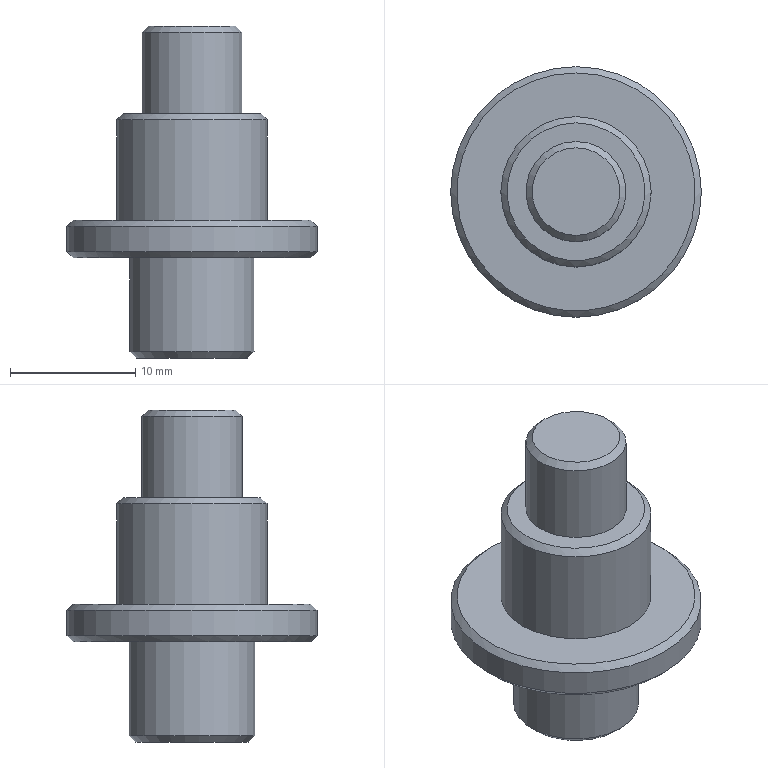Component | NX | SUPPORT_SHAFT | 1 solid | 14 faces | box 20 x 20 x 26.5 mm | volume 2857 mm3 | plane 5 | cone 5 | cylinder 4 | commonest cylinder face diameters 8 x1 12 x1 20 x1 10 x1
STEP:
#1=CARTESIAN_POINT('',(0.,0.,0.));
#2=DIRECTION('',(0.,0.,1.));
#3=DIRECTION('',(1.,0.,0.));
#4=AXIS2_PLACEMENT_3D('',#1,#2,#3);
#5=CARTESIAN_POINT('',(0.,3.5,3.5));
#6=VERTEX_POINT('',#5);
#7=CARTESIAN_POINT('',(0.,0.,3.5));
#8=DIRECTION('',(0.,0.,1.));
#9=DIRECTION('',(0.,1.,0.));
#10=AXIS2_PLACEMENT_3D('',#7,#8,#9);
#11=CIRCLE('',#10,3.5);
#12=CARTESIAN_POINT('',(0.,-4.,3.5));
#13=DIRECTION('',(0.,0.,-1.));
#14=DIRECTION('',(0.,1.,0.));
#15=AXIS2_PLACEMENT_3D('',#12,#13,#14);
#16=PLANE('',#15);
#17=CARTESIAN_POINT('',(7.5,0.));
#18=CARTESIAN_POINT('',(7.5,-6.062));
#19=CARTESIAN_POINT('',(2.25,-3.031));
#20=CARTESIAN_POINT('',(-3.,-0.));
#21=CARTESIAN_POINT('',(2.25,3.031));
#22=CARTESIAN_POINT('',(7.5,6.062));
#23=CARTESIAN_POINT('',(7.5,0.));
#24=(BOUNDED_CURVE()B_SPLINE_CURVE(2,(#17,#18,#19,#20,#21,#22,#23),.UNSPECIFIED.,.T.,.F.)B_SPLINE_CURVE_WITH_KNOTS((1,2,2,2,2,1),(-2.094,0.,2.094,4.189,6.283,8.378),.UNSPECIFIED.)CURVE()GEOMETRIC_REPRESENTATION_ITEM()RATIONAL_B_SPLINE_CURVE((1.,0.5,1.,0.5,1.,0.5,1.))REPRESENTATION_ITEM(''));
#25=(GEOMETRIC_REPRESENTATION_CONTEXT(2)PARAMETRIC_REPRESENTATION_CONTEXT()REPRESENTATION_CONTEXT('',''));
#26=DEFINITIONAL_REPRESENTATION('',(#24),#25);
#27=PCURVE('',#16,#26);
#28=CARTESIAN_POINT('',(0.,0.,3.5));
#29=DIRECTION('',(0.,0.,-1.));
#30=DIRECTION('',(0.,1.,0.));
#31=AXIS2_PLACEMENT_3D('',#28,#29,#30);
#32=CONICAL_SURFACE('',#31,3.5,0.7854);
#33=CARTESIAN_POINT('',(6.283,0.));
#34=DIRECTION('',(-1.,0.));
#35=VECTOR('',#34,1.);
#36=LINE('',#33,#35);
#37=(GEOMETRIC_REPRESENTATION_CONTEXT(2)PARAMETRIC_REPRESENTATION_CONTEXT()REPRESENTATION_CONTEXT('',''));
#38=DEFINITIONAL_REPRESENTATION('',(#36),#37);
#39=PCURVE('',#32,#38);
#40=SURFACE_CURVE('',#11,(#27,#39),.PCURVE_S1.);
#41=EDGE_CURVE('',#6,#6,#40,.T.);
#42=ORIENTED_EDGE('',*,*,#41,.T.);
#43=EDGE_LOOP('',(#42));
#44=FACE_BOUND('',#43,.T.);
#45=ADVANCED_FACE('',(#44),#16,.F.);
#46=CARTESIAN_POINT('',(0.,4.,3.));
#47=VERTEX_POINT('',#46);
#48=CARTESIAN_POINT('',(0.,-4.,3.));
#49=VERTEX_POINT('',#48);
#50=CARTESIAN_POINT('',(0.,0.,3.));
#51=DIRECTION('',(0.,0.,-1.));
#52=DIRECTION('',(0.,1.,0.));
#53=AXIS2_PLACEMENT_3D('',#50,#51,#52);
#54=CIRCLE('',#53,4.);
#55=CARTESIAN_POINT('',(0.,0.,-23.));
#56=DIRECTION('',(0.,0.,1.));
#57=DIRECTION('',(0.,-1.,0.));
#58=AXIS2_PLACEMENT_3D('',#55,#56,#57);
#59=CYLINDRICAL_SURFACE('',#58,4.);
#60=CARTESIAN_POINT('',(3.142,26.));
#61=DIRECTION('',(-1.,0.));
#62=VECTOR('',#61,1.);
#63=LINE('',#60,#62);
#64=(GEOMETRIC_REPRESENTATION_CONTEXT(2)PARAMETRIC_REPRESENTATION_CONTEXT()REPRESENTATION_CONTEXT('',''));
#65=DEFINITIONAL_REPRESENTATION('',(#63),#64);
#66=PCURVE('',#59,#65);
#67=CARTESIAN_POINT('',(0.,0.5));
#68=DIRECTION('',(1.,0.));
#69=VECTOR('',#68,1.);
#70=LINE('',#67,#69);
#71=(GEOMETRIC_REPRESENTATION_CONTEXT(2)PARAMETRIC_REPRESENTATION_CONTEXT()REPRESENTATION_CONTEXT('',''));
#72=DEFINITIONAL_REPRESENTATION('',(#70),#71);
#73=PCURVE('',#32,#72);
#74=SURFACE_CURVE('',#54,(#66,#73),.PCURVE_S1.);
#75=EDGE_CURVE('',#47,#49,#74,.T.);
#76=ORIENTED_EDGE('',*,*,#75,.T.);
#77=CARTESIAN_POINT('',(0.,-4.,-3.5));
#78=VERTEX_POINT('',#77);
#79=CARTESIAN_POINT('',(0.,-4.,-3.5));
#80=CARTESIAN_POINT('',(0.,-4.,3.));
#81=B_SPLINE_CURVE_WITH_KNOTS('',1,(#79,#80),.UNSPECIFIED.,.F.,.F.,(2,2),(19.5,26.),.PIECEWISE_BEZIER_KNOTS.);
#82=CARTESIAN_POINT('',(0.,0.));
#83=DIRECTION('',(0.,1.));
#84=VECTOR('',#83,1.);
#85=LINE('',#82,#84);
#86=(GEOMETRIC_REPRESENTATION_CONTEXT(2)PARAMETRIC_REPRESENTATION_CONTEXT()REPRESENTATION_CONTEXT('',''));
#87=DEFINITIONAL_REPRESENTATION('',(#85),#86);
#88=PCURVE('',#59,#87);
#89=CARTESIAN_POINT('',(6.283,0.));
#90=DIRECTION('',(0.,1.));
#91=VECTOR('',#90,1.);
#92=LINE('',#89,#91);
#93=(GEOMETRIC_REPRESENTATION_CONTEXT(2)PARAMETRIC_REPRESENTATION_CONTEXT()REPRESENTATION_CONTEXT('',''));
#94=DEFINITIONAL_REPRESENTATION('',(#92),#93);
#95=PCURVE('',#59,#94);
#96=SEAM_CURVE('',#81,(#88,#95),.PCURVE_S1.);
#97=EDGE_CURVE('',#78,#49,#96,.T.);
#98=ORIENTED_EDGE('',*,*,#97,.F.);
#99=CARTESIAN_POINT('',(0.,0.,-3.5));
#100=DIRECTION('',(0.,0.,1.));
#101=DIRECTION('',(0.,-1.,0.));
#102=AXIS2_PLACEMENT_3D('',#99,#100,#101);
#103=CIRCLE('',#102,4.);
#104=CARTESIAN_POINT('',(0.,19.5));
#105=DIRECTION('',(1.,0.));
#106=VECTOR('',#105,1.);
#107=LINE('',#104,#106);
#108=(GEOMETRIC_REPRESENTATION_CONTEXT(2)PARAMETRIC_REPRESENTATION_CONTEXT()REPRESENTATION_CONTEXT('',''));
#109=DEFINITIONAL_REPRESENTATION('',(#107),#108);
#110=PCURVE('',#59,#109);
#111=CARTESIAN_POINT('',(0.,-6.,-3.5));
#112=DIRECTION('',(0.,0.,-1.));
#113=DIRECTION('',(0.,1.,0.));
#114=AXIS2_PLACEMENT_3D('',#111,#112,#113);
#115=PLANE('',#114);
#116=CARTESIAN_POINT('',(2.,0.));
#117=CARTESIAN_POINT('',(2.,6.928));
#118=CARTESIAN_POINT('',(8.,3.464));
#119=CARTESIAN_POINT('',(14.,0.));
#120=CARTESIAN_POINT('',(8.,-3.464));
#121=CARTESIAN_POINT('',(2.,-6.928));
#122=CARTESIAN_POINT('',(2.,0.));
#123=(BOUNDED_CURVE()B_SPLINE_CURVE(2,(#116,#117,#118,#119,#120,#121,#122),.UNSPECIFIED.,.T.,.F.)B_SPLINE_CURVE_WITH_KNOTS((1,2,2,2,2,1),(-2.094,0.,2.094,4.189,6.283,8.378),.UNSPECIFIED.)CURVE()GEOMETRIC_REPRESENTATION_ITEM()RATIONAL_B_SPLINE_CURVE((1.,0.5,1.,0.5,1.,0.5,1.))REPRESENTATION_ITEM(''));
#124=(GEOMETRIC_REPRESENTATION_CONTEXT(2)PARAMETRIC_REPRESENTATION_CONTEXT()REPRESENTATION_CONTEXT('',''));
#125=DEFINITIONAL_REPRESENTATION('',(#123),#124);
#126=PCURVE('',#115,#125);
#127=SURFACE_CURVE('',#103,(#110,#126),.PCURVE_S1.);
#128=EDGE_CURVE('',#78,#78,#127,.T.);
#129=ORIENTED_EDGE('',*,*,#128,.T.);
#130=ORIENTED_EDGE('',*,*,#97,.T.);
#131=CARTESIAN_POINT('',(0.,0.,3.));
#132=DIRECTION('',(0.,0.,-1.));
#133=DIRECTION('',(0.,1.,0.));
#134=AXIS2_PLACEMENT_3D('',#131,#132,#133);
#135=CIRCLE('',#134,4.);
#136=CARTESIAN_POINT('',(9.425,26.));
#137=DIRECTION('',(-1.,0.));
#138=VECTOR('',#137,1.);
#139=LINE('',#136,#138);
#140=(GEOMETRIC_REPRESENTATION_CONTEXT(2)PARAMETRIC_REPRESENTATION_CONTEXT()REPRESENTATION_CONTEXT('',''));
#141=DEFINITIONAL_REPRESENTATION('',(#139),#140);
#142=PCURVE('',#59,#141);
#143=CARTESIAN_POINT('',(0.,0.5));
#144=DIRECTION('',(1.,0.));
#145=VECTOR('',#144,1.);
#146=LINE('',#143,#145);
#147=(GEOMETRIC_REPRESENTATION_CONTEXT(2)PARAMETRIC_REPRESENTATION_CONTEXT()REPRESENTATION_CONTEXT('',''));
#148=DEFINITIONAL_REPRESENTATION('',(#146),#147);
#149=PCURVE('',#32,#148);
#150=SURFACE_CURVE('',#135,(#142,#149),.PCURVE_S1.);
#151=EDGE_CURVE('',#49,#47,#150,.T.);
#152=ORIENTED_EDGE('',*,*,#151,.T.);
#153=EDGE_LOOP('',(#76,#98,#129,#130,#152));
#154=FACE_BOUND('',#153,.T.);
#155=ADVANCED_FACE('',(#154),#59,.T.);
#156=CARTESIAN_POINT('',(0.,5.5,-3.5));
#157=VERTEX_POINT('',#156);
#158=CARTESIAN_POINT('',(0.,0.,-3.5));
#159=DIRECTION('',(0.,0.,1.));
#160=DIRECTION('',(0.,1.,0.));
#161=AXIS2_PLACEMENT_3D('',#158,#159,#160);
#162=CIRCLE('',#161,5.5);
#163=CARTESIAN_POINT('',(11.5,0.));
#164=CARTESIAN_POINT('',(11.5,-9.526));
#165=CARTESIAN_POINT('',(3.25,-4.763));
#166=CARTESIAN_POINT('',(-5.,-0.));
#167=CARTESIAN_POINT('',(3.25,4.763));
#168=CARTESIAN_POINT('',(11.5,9.526));
#169=CARTESIAN_POINT('',(11.5,0.));
#170=(BOUNDED_CURVE()B_SPLINE_CURVE(2,(#163,#164,#165,#166,#167,#168,#169),.UNSPECIFIED.,.T.,.F.)B_SPLINE_CURVE_WITH_KNOTS((1,2,2,2,2,1),(-2.094,0.,2.094,4.189,6.283,8.378),.UNSPECIFIED.)CURVE()GEOMETRIC_REPRESENTATION_ITEM()RATIONAL_B_SPLINE_CURVE((1.,0.5,1.,0.5,1.,0.5,1.))REPRESENTATION_ITEM(''));
#171=(GEOMETRIC_REPRESENTATION_CONTEXT(2)PARAMETRIC_REPRESENTATION_CONTEXT()REPRESENTATION_CONTEXT('',''));
#172=DEFINITIONAL_REPRESENTATION('',(#170),#171);
#173=PCURVE('',#115,#172);
#174=CARTESIAN_POINT('',(0.,0.,-3.5));
#175=DIRECTION('',(0.,0.,-1.));
#176=DIRECTION('',(0.,1.,0.));
#177=AXIS2_PLACEMENT_3D('',#174,#175,#176);
#178=CONICAL_SURFACE('',#177,5.5,0.7854);
#179=CARTESIAN_POINT('',(6.283,0.));
#180=DIRECTION('',(-1.,0.));
#181=VECTOR('',#180,1.);
#182=LINE('',#179,#181);
#183=(GEOMETRIC_REPRESENTATION_CONTEXT(2)PARAMETRIC_REPRESENTATION_CONTEXT()REPRESENTATION_CONTEXT('',''));
#184=DEFINITIONAL_REPRESENTATION('',(#182),#183);
#185=PCURVE('',#178,#184);
#186=SURFACE_CURVE('',#162,(#173,#185),.PCURVE_S1.);
#187=EDGE_CURVE('',#157,#157,#186,.T.);
#188=ORIENTED_EDGE('',*,*,#187,.T.);
#189=EDGE_LOOP('',(#188));
#190=FACE_BOUND('',#189,.T.);
#191=ORIENTED_EDGE('',*,*,#128,.F.);
#192=EDGE_LOOP('',(#191));
#193=FACE_BOUND('',#192,.T.);
#194=ADVANCED_FACE('',(#190,#193),#115,.F.);
#195=CARTESIAN_POINT('',(0.,6.,-4.));
#196=VERTEX_POINT('',#195);
#197=CARTESIAN_POINT('',(0.,-6.,-4.));
#198=VERTEX_POINT('',#197);
#199=CARTESIAN_POINT('',(0.,0.,-4.));
#200=DIRECTION('',(0.,0.,-1.));
#201=DIRECTION('',(0.,1.,0.));
#202=AXIS2_PLACEMENT_3D('',#199,#200,#201);
#203=CIRCLE('',#202,6.);
#204=CARTESIAN_POINT('',(0.,0.,-23.));
#205=DIRECTION('',(0.,0.,1.));
#206=DIRECTION('',(0.,-1.,0.));
#207=AXIS2_PLACEMENT_3D('',#204,#205,#206);
#208=CYLINDRICAL_SURFACE('',#207,6.);
#209=CARTESIAN_POINT('',(3.142,19.));
#210=DIRECTION('',(-1.,0.));
#211=VECTOR('',#210,1.);
#212=LINE('',#209,#211);
#213=(GEOMETRIC_REPRESENTATION_CONTEXT(2)PARAMETRIC_REPRESENTATION_CONTEXT()REPRESENTATION_CONTEXT('',''));
#214=DEFINITIONAL_REPRESENTATION('',(#212),#213);
#215=PCURVE('',#208,#214);
#216=CARTESIAN_POINT('',(0.,0.5));
#217=DIRECTION('',(1.,0.));
#218=VECTOR('',#217,1.);
#219=LINE('',#216,#218);
#220=(GEOMETRIC_REPRESENTATION_CONTEXT(2)PARAMETRIC_REPRESENTATION_CONTEXT()REPRESENTATION_CONTEXT('',''));
#221=DEFINITIONAL_REPRESENTATION('',(#219),#220);
#222=PCURVE('',#178,#221);
#223=SURFACE_CURVE('',#203,(#215,#222),.PCURVE_S1.);
#224=EDGE_CURVE('',#196,#198,#223,.T.);
#225=ORIENTED_EDGE('',*,*,#224,.T.);
#226=CARTESIAN_POINT('',(0.,-6.,-12.));
#227=VERTEX_POINT('',#226);
#228=CARTESIAN_POINT('',(0.,-6.,-12.));
#229=CARTESIAN_POINT('',(0.,-6.,-4.));
#230=B_SPLINE_CURVE_WITH_KNOTS('',1,(#228,#229),.UNSPECIFIED.,.F.,.F.,(2,2),(11.,19.),.PIECEWISE_BEZIER_KNOTS.);
#231=CARTESIAN_POINT('',(0.,0.));
#232=DIRECTION('',(0.,1.));
#233=VECTOR('',#232,1.);
#234=LINE('',#231,#233);
#235=(GEOMETRIC_REPRESENTATION_CONTEXT(2)PARAMETRIC_REPRESENTATION_CONTEXT()REPRESENTATION_CONTEXT('',''));
#236=DEFINITIONAL_REPRESENTATION('',(#234),#235);
#237=PCURVE('',#208,#236);
#238=CARTESIAN_POINT('',(6.283,0.));
#239=DIRECTION('',(0.,1.));
#240=VECTOR('',#239,1.);
#241=LINE('',#238,#240);
#242=(GEOMETRIC_REPRESENTATION_CONTEXT(2)PARAMETRIC_REPRESENTATION_CONTEXT()REPRESENTATION_CONTEXT('',''));
#243=DEFINITIONAL_REPRESENTATION('',(#241),#242);
#244=PCURVE('',#208,#243);
#245=SEAM_CURVE('',#230,(#237,#244),.PCURVE_S1.);
#246=EDGE_CURVE('',#227,#198,#245,.T.);
#247=ORIENTED_EDGE('',*,*,#246,.F.);
#248=CARTESIAN_POINT('',(0.,0.,-12.));
#249=DIRECTION('',(0.,0.,1.));
#250=DIRECTION('',(0.,-1.,0.));
#251=AXIS2_PLACEMENT_3D('',#248,#249,#250);
#252=CIRCLE('',#251,6.);
#253=CARTESIAN_POINT('',(0.,11.));
#254=DIRECTION('',(1.,0.));
#255=VECTOR('',#254,1.);
#256=LINE('',#253,#255);
#257=(GEOMETRIC_REPRESENTATION_CONTEXT(2)PARAMETRIC_REPRESENTATION_CONTEXT()REPRESENTATION_CONTEXT('',''));
#258=DEFINITIONAL_REPRESENTATION('',(#256),#257);
#259=PCURVE('',#208,#258);
#260=CARTESIAN_POINT('',(0.,-10.,-12.));
#261=DIRECTION('',(0.,0.,-1.));
#262=DIRECTION('',(0.,1.,0.));
#263=AXIS2_PLACEMENT_3D('',#260,#261,#262);
#264=PLANE('',#263);
#265=CARTESIAN_POINT('',(4.,0.));
#266=CARTESIAN_POINT('',(4.,10.392));
#267=CARTESIAN_POINT('',(13.,5.196));
#268=CARTESIAN_POINT('',(22.,0.));
#269=CARTESIAN_POINT('',(13.,-5.196));
#270=CARTESIAN_POINT('',(4.,-10.392));
#271=CARTESIAN_POINT('',(4.,0.));
#272=(BOUNDED_CURVE()B_SPLINE_CURVE(2,(#265,#266,#267,#268,#269,#270,#271),.UNSPECIFIED.,.T.,.F.)B_SPLINE_CURVE_WITH_KNOTS((1,2,2,2,2,1),(-2.094,0.,2.094,4.189,6.283,8.378),.UNSPECIFIED.)CURVE()GEOMETRIC_REPRESENTATION_ITEM()RATIONAL_B_SPLINE_CURVE((1.,0.5,1.,0.5,1.,0.5,1.))REPRESENTATION_ITEM(''));
#273=(GEOMETRIC_REPRESENTATION_CONTEXT(2)PARAMETRIC_REPRESENTATION_CONTEXT()REPRESENTATION_CONTEXT('',''));
#274=DEFINITIONAL_REPRESENTATION('',(#272),#273);
#275=PCURVE('',#264,#274);
#276=SURFACE_CURVE('',#252,(#259,#275),.PCURVE_S1.);
#277=EDGE_CURVE('',#227,#227,#276,.T.);
#278=ORIENTED_EDGE('',*,*,#277,.T.);
#279=ORIENTED_EDGE('',*,*,#246,.T.);
#280=CARTESIAN_POINT('',(0.,0.,-4.));
#281=DIRECTION('',(0.,0.,-1.));
#282=DIRECTION('',(0.,1.,0.));
#283=AXIS2_PLACEMENT_3D('',#280,#281,#282);
#284=CIRCLE('',#283,6.);
#285=CARTESIAN_POINT('',(9.425,19.));
#286=DIRECTION('',(-1.,0.));
#287=VECTOR('',#286,1.);
#288=LINE('',#285,#287);
#289=(GEOMETRIC_REPRESENTATION_CONTEXT(2)PARAMETRIC_REPRESENTATION_CONTEXT()REPRESENTATION_CONTEXT('',''));
#290=DEFINITIONAL_REPRESENTATION('',(#288),#289);
#291=PCURVE('',#208,#290);
#292=CARTESIAN_POINT('',(0.,0.5));
#293=DIRECTION('',(1.,0.));
#294=VECTOR('',#293,1.);
#295=LINE('',#292,#294);
#296=(GEOMETRIC_REPRESENTATION_CONTEXT(2)PARAMETRIC_REPRESENTATION_CONTEXT()REPRESENTATION_CONTEXT('',''));
#297=DEFINITIONAL_REPRESENTATION('',(#295),#296);
#298=PCURVE('',#178,#297);
#299=SURFACE_CURVE('',#284,(#291,#298),.PCURVE_S1.);
#300=EDGE_CURVE('',#198,#196,#299,.T.);
#301=ORIENTED_EDGE('',*,*,#300,.T.);
#302=EDGE_LOOP('',(#225,#247,#278,#279,#301));
#303=FACE_BOUND('',#302,.T.);
#304=ADVANCED_FACE('',(#303),#208,.T.);
#305=CARTESIAN_POINT('',(0.,9.5,-12.));
#306=VERTEX_POINT('',#305);
#307=CARTESIAN_POINT('',(0.,0.,-12.));
#308=DIRECTION('',(0.,0.,1.));
#309=DIRECTION('',(0.,1.,0.));
#310=AXIS2_PLACEMENT_3D('',#307,#308,#309);
#311=CIRCLE('',#310,9.5);
#312=CARTESIAN_POINT('',(19.5,0.));
#313=CARTESIAN_POINT('',(19.5,-16.454));
#314=CARTESIAN_POINT('',(5.25,-8.227));
#315=CARTESIAN_POINT('',(-9.,-0.));
#316=CARTESIAN_POINT('',(5.25,8.227));
#317=CARTESIAN_POINT('',(19.5,16.454));
#318=CARTESIAN_POINT('',(19.5,0.));
#319=(BOUNDED_CURVE()B_SPLINE_CURVE(2,(#312,#313,#314,#315,#316,#317,#318),.UNSPECIFIED.,.T.,.F.)B_SPLINE_CURVE_WITH_KNOTS((1,2,2,2,2,1),(-2.094,0.,2.094,4.189,6.283,8.378),.UNSPECIFIED.)CURVE()GEOMETRIC_REPRESENTATION_ITEM()RATIONAL_B_SPLINE_CURVE((1.,0.5,1.,0.5,1.,0.5,1.))REPRESENTATION_ITEM(''));
#320=(GEOMETRIC_REPRESENTATION_CONTEXT(2)PARAMETRIC_REPRESENTATION_CONTEXT()REPRESENTATION_CONTEXT('',''));
#321=DEFINITIONAL_REPRESENTATION('',(#319),#320);
#322=PCURVE('',#264,#321);
#323=CARTESIAN_POINT('',(0.,0.,-12.));
#324=DIRECTION('',(0.,0.,-1.));
#325=DIRECTION('',(0.,1.,0.));
#326=AXIS2_PLACEMENT_3D('',#323,#324,#325);
#327=CONICAL_SURFACE('',#326,9.5,0.7854);
#328=CARTESIAN_POINT('',(6.283,0.));
#329=DIRECTION('',(-1.,0.));
#330=VECTOR('',#329,1.);
#331=LINE('',#328,#330);
#332=(GEOMETRIC_REPRESENTATION_CONTEXT(2)PARAMETRIC_REPRESENTATION_CONTEXT()REPRESENTATION_CONTEXT('',''));
#333=DEFINITIONAL_REPRESENTATION('',(#331),#332);
#334=PCURVE('',#327,#333);
#335=SURFACE_CURVE('',#311,(#322,#334),.PCURVE_S1.);
#336=EDGE_CURVE('',#306,#306,#335,.T.);
#337=ORIENTED_EDGE('',*,*,#336,.T.);
#338=EDGE_LOOP('',(#337));
#339=FACE_BOUND('',#338,.T.);
#340=ORIENTED_EDGE('',*,*,#277,.F.);
#341=EDGE_LOOP('',(#340));
#342=FACE_BOUND('',#341,.T.);
#343=ADVANCED_FACE('',(#339,#342),#264,.F.);
#344=CARTESIAN_POINT('',(0.,10.,-12.5));
#345=VERTEX_POINT('',#344);
#346=CARTESIAN_POINT('',(0.,-10.,-12.5));
#347=VERTEX_POINT('',#346);
#348=CARTESIAN_POINT('',(0.,0.,-12.5));
#349=DIRECTION('',(0.,0.,-1.));
#350=DIRECTION('',(0.,1.,0.));
#351=AXIS2_PLACEMENT_3D('',#348,#349,#350);
#352=CIRCLE('',#351,10.);
#353=CARTESIAN_POINT('',(0.,0.,-23.));
#354=DIRECTION('',(0.,0.,1.));
#355=DIRECTION('',(0.,-1.,0.));
#356=AXIS2_PLACEMENT_3D('',#353,#354,#355);
#357=CYLINDRICAL_SURFACE('',#356,10.);
#358=CARTESIAN_POINT('',(3.142,10.5));
#359=DIRECTION('',(-1.,0.));
#360=VECTOR('',#359,1.);
#361=LINE('',#358,#360);
#362=(GEOMETRIC_REPRESENTATION_CONTEXT(2)PARAMETRIC_REPRESENTATION_CONTEXT()REPRESENTATION_CONTEXT('',''));
#363=DEFINITIONAL_REPRESENTATION('',(#361),#362);
#364=PCURVE('',#357,#363);
#365=CARTESIAN_POINT('',(0.,0.5));
#366=DIRECTION('',(1.,0.));
#367=VECTOR('',#366,1.);
#368=LINE('',#365,#367);
#369=(GEOMETRIC_REPRESENTATION_CONTEXT(2)PARAMETRIC_REPRESENTATION_CONTEXT()REPRESENTATION_CONTEXT('',''));
#370=DEFINITIONAL_REPRESENTATION('',(#368),#369);
#371=PCURVE('',#327,#370);
#372=SURFACE_CURVE('',#352,(#364,#371),.PCURVE_S1.);
#373=EDGE_CURVE('',#345,#347,#372,.T.);
#374=ORIENTED_EDGE('',*,*,#373,.T.);
#375=CARTESIAN_POINT('',(0.,-10.,-14.5));
#376=VERTEX_POINT('',#375);
#377=CARTESIAN_POINT('',(0.,-10.,-14.5));
#378=CARTESIAN_POINT('',(0.,-10.,-12.5));
#379=B_SPLINE_CURVE_WITH_KNOTS('',1,(#377,#378),.UNSPECIFIED.,.F.,.F.,(2,2),(8.5,10.5),.PIECEWISE_BEZIER_KNOTS.);
#380=CARTESIAN_POINT('',(0.,0.));
#381=DIRECTION('',(0.,1.));
#382=VECTOR('',#381,1.);
#383=LINE('',#380,#382);
#384=(GEOMETRIC_REPRESENTATION_CONTEXT(2)PARAMETRIC_REPRESENTATION_CONTEXT()REPRESENTATION_CONTEXT('',''));
#385=DEFINITIONAL_REPRESENTATION('',(#383),#384);
#386=PCURVE('',#357,#385);
#387=CARTESIAN_POINT('',(6.283,0.));
#388=DIRECTION('',(0.,1.));
#389=VECTOR('',#388,1.);
#390=LINE('',#387,#389);
#391=(GEOMETRIC_REPRESENTATION_CONTEXT(2)PARAMETRIC_REPRESENTATION_CONTEXT()REPRESENTATION_CONTEXT('',''));
#392=DEFINITIONAL_REPRESENTATION('',(#390),#391);
#393=PCURVE('',#357,#392);
#394=SEAM_CURVE('',#379,(#386,#393),.PCURVE_S1.);
#395=EDGE_CURVE('',#376,#347,#394,.T.);
#396=ORIENTED_EDGE('',*,*,#395,.F.);
#397=CARTESIAN_POINT('',(0.,0.,-14.5));
#398=DIRECTION('',(0.,0.,1.));
#399=DIRECTION('',(0.,-1.,0.));
#400=AXIS2_PLACEMENT_3D('',#397,#398,#399);
#401=CIRCLE('',#400,10.);
#402=CARTESIAN_POINT('',(0.,8.5));
#403=DIRECTION('',(1.,0.));
#404=VECTOR('',#403,1.);
#405=LINE('',#402,#404);
#406=(GEOMETRIC_REPRESENTATION_CONTEXT(2)PARAMETRIC_REPRESENTATION_CONTEXT()REPRESENTATION_CONTEXT('',''));
#407=DEFINITIONAL_REPRESENTATION('',(#405),#406);
#408=PCURVE('',#357,#407);
#409=CARTESIAN_POINT('',(0.,0.,-14.5));
#410=DIRECTION('',(0.,0.,1.));
#411=DIRECTION('',(0.,-1.,0.));
#412=AXIS2_PLACEMENT_3D('',#409,#410,#411);
#413=CONICAL_SURFACE('',#412,10.,0.7854);
#414=CARTESIAN_POINT('',(0.,0.));
#415=DIRECTION('',(1.,0.));
#416=VECTOR('',#415,1.);
#417=LINE('',#414,#416);
#418=(GEOMETRIC_REPRESENTATION_CONTEXT(2)PARAMETRIC_REPRESENTATION_CONTEXT()REPRESENTATION_CONTEXT('',''));
#419=DEFINITIONAL_REPRESENTATION('',(#417),#418);
#420=PCURVE('',#413,#419);
#421=SURFACE_CURVE('',#401,(#408,#420),.PCURVE_S1.);
#422=EDGE_CURVE('',#376,#376,#421,.T.);
#423=ORIENTED_EDGE('',*,*,#422,.T.);
#424=ORIENTED_EDGE('',*,*,#395,.T.);
#425=CARTESIAN_POINT('',(0.,0.,-12.5));
#426=DIRECTION('',(0.,0.,-1.));
#427=DIRECTION('',(0.,1.,0.));
#428=AXIS2_PLACEMENT_3D('',#425,#426,#427);
#429=CIRCLE('',#428,10.);
#430=CARTESIAN_POINT('',(9.425,10.5));
#431=DIRECTION('',(-1.,0.));
#432=VECTOR('',#431,1.);
#433=LINE('',#430,#432);
#434=(GEOMETRIC_REPRESENTATION_CONTEXT(2)PARAMETRIC_REPRESENTATION_CONTEXT()REPRESENTATION_CONTEXT('',''));
#435=DEFINITIONAL_REPRESENTATION('',(#433),#434);
#436=PCURVE('',#357,#435);
#437=CARTESIAN_POINT('',(0.,0.5));
#438=DIRECTION('',(1.,0.));
#439=VECTOR('',#438,1.);
#440=LINE('',#437,#439);
#441=(GEOMETRIC_REPRESENTATION_CONTEXT(2)PARAMETRIC_REPRESENTATION_CONTEXT()REPRESENTATION_CONTEXT('',''));
#442=DEFINITIONAL_REPRESENTATION('',(#440),#441);
#443=PCURVE('',#327,#442);
#444=SURFACE_CURVE('',#429,(#436,#443),.PCURVE_S1.);
#445=EDGE_CURVE('',#347,#345,#444,.T.);
#446=ORIENTED_EDGE('',*,*,#445,.T.);
#447=EDGE_LOOP('',(#374,#396,#423,#424,#446));
#448=FACE_BOUND('',#447,.T.);
#449=ADVANCED_FACE('',(#448),#357,.T.);
#450=CARTESIAN_POINT('',(0.,-9.5,-15.));
#451=VERTEX_POINT('',#450);
#452=CARTESIAN_POINT('',(0.,0.,-15.));
#453=DIRECTION('',(0.,0.,-1.));
#454=DIRECTION('',(0.,-1.,0.));
#455=AXIS2_PLACEMENT_3D('',#452,#453,#454);
#456=CIRCLE('',#455,9.5);
#457=CARTESIAN_POINT('',(0.,-5.,-15.));
#458=DIRECTION('',(0.,0.,1.));
#459=DIRECTION('',(0.,-1.,0.));
#460=AXIS2_PLACEMENT_3D('',#457,#458,#459);
#461=PLANE('',#460);
#462=CARTESIAN_POINT('',(4.5,0.));
#463=CARTESIAN_POINT('',(4.5,-16.454));
#464=CARTESIAN_POINT('',(-9.75,-8.227));
#465=CARTESIAN_POINT('',(-24.,-0.));
#466=CARTESIAN_POINT('',(-9.75,8.227));
#467=CARTESIAN_POINT('',(4.5,16.454));
#468=CARTESIAN_POINT('',(4.5,0.));
#469=(BOUNDED_CURVE()B_SPLINE_CURVE(2,(#462,#463,#464,#465,#466,#467,#468),.UNSPECIFIED.,.T.,.F.)B_SPLINE_CURVE_WITH_KNOTS((1,2,2,2,2,1),(-2.094,0.,2.094,4.189,6.283,8.378),.UNSPECIFIED.)CURVE()GEOMETRIC_REPRESENTATION_ITEM()RATIONAL_B_SPLINE_CURVE((1.,0.5,1.,0.5,1.,0.5,1.))REPRESENTATION_ITEM(''));
#470=(GEOMETRIC_REPRESENTATION_CONTEXT(2)PARAMETRIC_REPRESENTATION_CONTEXT()REPRESENTATION_CONTEXT('',''));
#471=DEFINITIONAL_REPRESENTATION('',(#469),#470);
#472=PCURVE('',#461,#471);
#473=CARTESIAN_POINT('',(6.283,-0.5));
#474=DIRECTION('',(-1.,0.));
#475=VECTOR('',#474,1.);
#476=LINE('',#473,#475);
#477=(GEOMETRIC_REPRESENTATION_CONTEXT(2)PARAMETRIC_REPRESENTATION_CONTEXT()REPRESENTATION_CONTEXT('',''));
#478=DEFINITIONAL_REPRESENTATION('',(#476),#477);
#479=PCURVE('',#413,#478);
#480=SURFACE_CURVE('',#456,(#472,#479),.PCURVE_S1.);
#481=EDGE_CURVE('',#451,#451,#480,.T.);
#482=ORIENTED_EDGE('',*,*,#481,.T.);
#483=EDGE_LOOP('',(#482));
#484=FACE_BOUND('',#483,.T.);
#485=CARTESIAN_POINT('',(0.,-5.,-15.));
#486=VERTEX_POINT('',#485);
#487=CARTESIAN_POINT('',(0.,0.,-15.));
#488=DIRECTION('',(0.,0.,1.));
#489=DIRECTION('',(0.,-1.,0.));
#490=AXIS2_PLACEMENT_3D('',#487,#488,#489);
#491=CIRCLE('',#490,5.);
#492=CARTESIAN_POINT('',(-5.,0.));
#493=DIRECTION('',(1.,0.));
#494=AXIS2_PLACEMENT_2D('',#492,#493);
#495=CIRCLE('',#494,5.);
#496=(GEOMETRIC_REPRESENTATION_CONTEXT(2)PARAMETRIC_REPRESENTATION_CONTEXT()REPRESENTATION_CONTEXT('',''));
#497=DEFINITIONAL_REPRESENTATION('',(#495),#496);
#498=PCURVE('',#461,#497);
#499=CARTESIAN_POINT('',(0.,0.,-23.));
#500=DIRECTION('',(0.,0.,1.));
#501=DIRECTION('',(0.,-1.,0.));
#502=AXIS2_PLACEMENT_3D('',#499,#500,#501);
#503=CYLINDRICAL_SURFACE('',#502,5.);
#504=CARTESIAN_POINT('',(0.,8.));
#505=DIRECTION('',(1.,0.));
#506=VECTOR('',#505,1.);
#507=LINE('',#504,#506);
#508=(GEOMETRIC_REPRESENTATION_CONTEXT(2)PARAMETRIC_REPRESENTATION_CONTEXT()REPRESENTATION_CONTEXT('',''));
#509=DEFINITIONAL_REPRESENTATION('',(#507),#508);
#510=PCURVE('',#503,#509);
#511=SURFACE_CURVE('',#491,(#498,#510),.PCURVE_S1.);
#512=EDGE_CURVE('',#486,#486,#511,.T.);
#513=ORIENTED_EDGE('',*,*,#512,.T.);
#514=EDGE_LOOP('',(#513));
#515=FACE_BOUND('',#514,.T.);
#516=ADVANCED_FACE('',(#484,#515),#461,.F.);
#517=CARTESIAN_POINT('',(0.,-5.,-22.5));
#518=VERTEX_POINT('',#517);
#519=CARTESIAN_POINT('',(0.,0.,-22.5));
#520=DIRECTION('',(0.,0.,1.));
#521=DIRECTION('',(0.,-1.,0.));
#522=AXIS2_PLACEMENT_3D('',#519,#520,#521);
#523=CIRCLE('',#522,5.);
#524=CARTESIAN_POINT('',(0.,0.5));
#525=DIRECTION('',(1.,0.));
#526=VECTOR('',#525,1.);
#527=LINE('',#524,#526);
#528=(GEOMETRIC_REPRESENTATION_CONTEXT(2)PARAMETRIC_REPRESENTATION_CONTEXT()REPRESENTATION_CONTEXT('',''));
#529=DEFINITIONAL_REPRESENTATION('',(#527),#528);
#530=PCURVE('',#503,#529);
#531=CARTESIAN_POINT('',(0.,0.,-22.5));
#532=DIRECTION('',(0.,0.,1.));
#533=DIRECTION('',(0.,-1.,0.));
#534=AXIS2_PLACEMENT_3D('',#531,#532,#533);
#535=CONICAL_SURFACE('',#534,5.,0.7854);
#536=CARTESIAN_POINT('',(0.,0.));
#537=DIRECTION('',(1.,0.));
#538=VECTOR('',#537,1.);
#539=LINE('',#536,#538);
#540=(GEOMETRIC_REPRESENTATION_CONTEXT(2)PARAMETRIC_REPRESENTATION_CONTEXT()REPRESENTATION_CONTEXT('',''));
#541=DEFINITIONAL_REPRESENTATION('',(#539),#540);
#542=PCURVE('',#535,#541);
#543=SURFACE_CURVE('',#523,(#530,#542),.PCURVE_S1.);
#544=EDGE_CURVE('',#518,#518,#543,.T.);
#545=ORIENTED_EDGE('',*,*,#544,.T.);
#546=CARTESIAN_POINT('',(0.,-5.,-22.5));
#547=CARTESIAN_POINT('',(0.,-5.,-15.));
#548=B_SPLINE_CURVE_WITH_KNOTS('',1,(#546,#547),.UNSPECIFIED.,.F.,.F.,(2,2),(0.5,8.),.PIECEWISE_BEZIER_KNOTS.);
#549=CARTESIAN_POINT('',(6.283,0.));
#550=DIRECTION('',(0.,1.));
#551=VECTOR('',#550,1.);
#552=LINE('',#549,#551);
#553=(GEOMETRIC_REPRESENTATION_CONTEXT(2)PARAMETRIC_REPRESENTATION_CONTEXT()REPRESENTATION_CONTEXT('',''));
#554=DEFINITIONAL_REPRESENTATION('',(#552),#553);
#555=PCURVE('',#503,#554);
#556=CARTESIAN_POINT('',(0.,0.));
#557=DIRECTION('',(0.,1.));
#558=VECTOR('',#557,1.);
#559=LINE('',#556,#558);
#560=(GEOMETRIC_REPRESENTATION_CONTEXT(2)PARAMETRIC_REPRESENTATION_CONTEXT()REPRESENTATION_CONTEXT('',''));
#561=DEFINITIONAL_REPRESENTATION('',(#559),#560);
#562=PCURVE('',#503,#561);
#563=SEAM_CURVE('',#548,(#555,#562),.PCURVE_S1.);
#564=EDGE_CURVE('',#518,#486,#563,.T.);
#565=ORIENTED_EDGE('',*,*,#564,.T.);
#566=ORIENTED_EDGE('',*,*,#512,.F.);
#567=ORIENTED_EDGE('',*,*,#564,.F.);
#568=EDGE_LOOP('',(#545,#565,#566,#567));
#569=FACE_BOUND('',#568,.T.);
#570=ADVANCED_FACE('',(#569),#503,.T.);
#571=CARTESIAN_POINT('',(0.,-4.5,-23.));
#572=VERTEX_POINT('',#571);
#573=CARTESIAN_POINT('',(0.,0.,-23.));
#574=DIRECTION('',(0.,0.,-1.));
#575=DIRECTION('',(0.,-1.,0.));
#576=AXIS2_PLACEMENT_3D('',#573,#574,#575);
#577=CIRCLE('',#576,4.5);
#578=CARTESIAN_POINT('',(0.,0.,-23.));
#579=DIRECTION('',(0.,0.,1.));
#580=DIRECTION('',(0.,-1.,0.));
#581=AXIS2_PLACEMENT_3D('',#578,#579,#580);
#582=PLANE('',#581);
#583=CARTESIAN_POINT('',(4.5,0.));
#584=CARTESIAN_POINT('',(4.5,-7.794));
#585=CARTESIAN_POINT('',(-2.25,-3.897));
#586=CARTESIAN_POINT('',(-9.,-0.));
#587=CARTESIAN_POINT('',(-2.25,3.897));
#588=CARTESIAN_POINT('',(4.5,7.794));
#589=CARTESIAN_POINT('',(4.5,0.));
#590=(BOUNDED_CURVE()B_SPLINE_CURVE(2,(#583,#584,#585,#586,#587,#588,#589),.UNSPECIFIED.,.T.,.F.)B_SPLINE_CURVE_WITH_KNOTS((1,2,2,2,2,1),(-2.094,0.,2.094,4.189,6.283,8.378),.UNSPECIFIED.)CURVE()GEOMETRIC_REPRESENTATION_ITEM()RATIONAL_B_SPLINE_CURVE((1.,0.5,1.,0.5,1.,0.5,1.))REPRESENTATION_ITEM(''));
#591=(GEOMETRIC_REPRESENTATION_CONTEXT(2)PARAMETRIC_REPRESENTATION_CONTEXT()REPRESENTATION_CONTEXT('',''));
#592=DEFINITIONAL_REPRESENTATION('',(#590),#591);
#593=PCURVE('',#582,#592);
#594=CARTESIAN_POINT('',(6.283,-0.5));
#595=DIRECTION('',(-1.,0.));
#596=VECTOR('',#595,1.);
#597=LINE('',#594,#596);
#598=(GEOMETRIC_REPRESENTATION_CONTEXT(2)PARAMETRIC_REPRESENTATION_CONTEXT()REPRESENTATION_CONTEXT('',''));
#599=DEFINITIONAL_REPRESENTATION('',(#597),#598);
#600=PCURVE('',#535,#599);
#601=SURFACE_CURVE('',#577,(#593,#600),.PCURVE_S1.);
#602=EDGE_CURVE('',#572,#572,#601,.T.);
#603=ORIENTED_EDGE('',*,*,#602,.T.);
#604=EDGE_LOOP('',(#603));
#605=FACE_BOUND('',#604,.T.);
#606=ADVANCED_FACE('',(#605),#582,.F.);
#607=ORIENTED_EDGE('',*,*,#602,.F.);
#608=CARTESIAN_POINT('',(0.,-4.5,-23.));
#609=CARTESIAN_POINT('',(0.,-5.,-22.5));
#610=B_SPLINE_CURVE_WITH_KNOTS('',1,(#608,#609),.UNSPECIFIED.,.F.,.F.,(2,2),(-0.7071,0.),.PIECEWISE_BEZIER_KNOTS.);
#611=CARTESIAN_POINT('',(6.283,0.));
#612=DIRECTION('',(0.,1.));
#613=VECTOR('',#612,1.);
#614=LINE('',#611,#613);
#615=(GEOMETRIC_REPRESENTATION_CONTEXT(2)PARAMETRIC_REPRESENTATION_CONTEXT()REPRESENTATION_CONTEXT('',''));
#616=DEFINITIONAL_REPRESENTATION('',(#614),#615);
#617=PCURVE('',#535,#616);
#618=CARTESIAN_POINT('',(0.,0.));
#619=DIRECTION('',(0.,1.));
#620=VECTOR('',#619,1.);
#621=LINE('',#618,#620);
#622=(GEOMETRIC_REPRESENTATION_CONTEXT(2)PARAMETRIC_REPRESENTATION_CONTEXT()REPRESENTATION_CONTEXT('',''));
#623=DEFINITIONAL_REPRESENTATION('',(#621),#622);
#624=PCURVE('',#535,#623);
#625=SEAM_CURVE('',#610,(#617,#624),.PCURVE_S1.);
#626=EDGE_CURVE('',#572,#518,#625,.T.);
#627=ORIENTED_EDGE('',*,*,#626,.T.);
#628=ORIENTED_EDGE('',*,*,#544,.F.);
#629=ORIENTED_EDGE('',*,*,#626,.F.);
#630=EDGE_LOOP('',(#607,#627,#628,#629));
#631=FACE_BOUND('',#630,.T.);
#632=ADVANCED_FACE('',(#631),#535,.T.);
#633=ORIENTED_EDGE('',*,*,#75,.F.);
#634=CARTESIAN_POINT('',(0.,3.5,3.5));
#635=CARTESIAN_POINT('',(0.,4.,3.));
#636=B_SPLINE_CURVE_WITH_KNOTS('',1,(#634,#635),.UNSPECIFIED.,.F.,.F.,(2,2),(0.,0.7071),.PIECEWISE_BEZIER_KNOTS.);
#637=CARTESIAN_POINT('',(0.,0.));
#638=DIRECTION('',(0.,1.));
#639=VECTOR('',#638,1.);
#640=LINE('',#637,#639);
#641=(GEOMETRIC_REPRESENTATION_CONTEXT(2)PARAMETRIC_REPRESENTATION_CONTEXT()REPRESENTATION_CONTEXT('',''));
#642=DEFINITIONAL_REPRESENTATION('',(#640),#641);
#643=PCURVE('',#32,#642);
#644=CARTESIAN_POINT('',(6.283,0.));
#645=DIRECTION('',(0.,1.));
#646=VECTOR('',#645,1.);
#647=LINE('',#644,#646);
#648=(GEOMETRIC_REPRESENTATION_CONTEXT(2)PARAMETRIC_REPRESENTATION_CONTEXT()REPRESENTATION_CONTEXT('',''));
#649=DEFINITIONAL_REPRESENTATION('',(#647),#648);
#650=PCURVE('',#32,#649);
#651=SEAM_CURVE('',#636,(#643,#650),.PCURVE_S1.);
#652=EDGE_CURVE('',#6,#47,#651,.T.);
#653=ORIENTED_EDGE('',*,*,#652,.F.);
#654=ORIENTED_EDGE('',*,*,#41,.F.);
#655=ORIENTED_EDGE('',*,*,#652,.T.);
#656=ORIENTED_EDGE('',*,*,#151,.F.);
#657=EDGE_LOOP('',(#633,#653,#654,#655,#656));
#658=FACE_BOUND('',#657,.T.);
#659=ADVANCED_FACE('',(#658),#32,.T.);
#660=ORIENTED_EDGE('',*,*,#224,.F.);
#661=CARTESIAN_POINT('',(0.,5.5,-3.5));
#662=CARTESIAN_POINT('',(0.,6.,-4.));
#663=B_SPLINE_CURVE_WITH_KNOTS('',1,(#661,#662),.UNSPECIFIED.,.F.,.F.,(2,2),(0.,0.7071),.PIECEWISE_BEZIER_KNOTS.);
#664=CARTESIAN_POINT('',(0.,0.));
#665=DIRECTION('',(0.,1.));
#666=VECTOR('',#665,1.);
#667=LINE('',#664,#666);
#668=(GEOMETRIC_REPRESENTATION_CONTEXT(2)PARAMETRIC_REPRESENTATION_CONTEXT()REPRESENTATION_CONTEXT('',''));
#669=DEFINITIONAL_REPRESENTATION('',(#667),#668);
#670=PCURVE('',#178,#669);
#671=CARTESIAN_POINT('',(6.283,0.));
#672=DIRECTION('',(0.,1.));
#673=VECTOR('',#672,1.);
#674=LINE('',#671,#673);
#675=(GEOMETRIC_REPRESENTATION_CONTEXT(2)PARAMETRIC_REPRESENTATION_CONTEXT()REPRESENTATION_CONTEXT('',''));
#676=DEFINITIONAL_REPRESENTATION('',(#674),#675);
#677=PCURVE('',#178,#676);
#678=SEAM_CURVE('',#663,(#670,#677),.PCURVE_S1.);
#679=EDGE_CURVE('',#157,#196,#678,.T.);
#680=ORIENTED_EDGE('',*,*,#679,.F.);
#681=ORIENTED_EDGE('',*,*,#187,.F.);
#682=ORIENTED_EDGE('',*,*,#679,.T.);
#683=ORIENTED_EDGE('',*,*,#300,.F.);
#684=EDGE_LOOP('',(#660,#680,#681,#682,#683));
#685=FACE_BOUND('',#684,.T.);
#686=ADVANCED_FACE('',(#685),#178,.T.);
#687=ORIENTED_EDGE('',*,*,#373,.F.);
#688=CARTESIAN_POINT('',(0.,9.5,-12.));
#689=CARTESIAN_POINT('',(0.,10.,-12.5));
#690=B_SPLINE_CURVE_WITH_KNOTS('',1,(#688,#689),.UNSPECIFIED.,.F.,.F.,(2,2),(0.,0.7071),.PIECEWISE_BEZIER_KNOTS.);
#691=CARTESIAN_POINT('',(0.,0.));
#692=DIRECTION('',(0.,1.));
#693=VECTOR('',#692,1.);
#694=LINE('',#691,#693);
#695=(GEOMETRIC_REPRESENTATION_CONTEXT(2)PARAMETRIC_REPRESENTATION_CONTEXT()REPRESENTATION_CONTEXT('',''));
#696=DEFINITIONAL_REPRESENTATION('',(#694),#695);
#697=PCURVE('',#327,#696);
#698=CARTESIAN_POINT('',(6.283,0.));
#699=DIRECTION('',(0.,1.));
#700=VECTOR('',#699,1.);
#701=LINE('',#698,#700);
#702=(GEOMETRIC_REPRESENTATION_CONTEXT(2)PARAMETRIC_REPRESENTATION_CONTEXT()REPRESENTATION_CONTEXT('',''));
#703=DEFINITIONAL_REPRESENTATION('',(#701),#702);
#704=PCURVE('',#327,#703);
#705=SEAM_CURVE('',#690,(#697,#704),.PCURVE_S1.);
#706=EDGE_CURVE('',#306,#345,#705,.T.);
#707=ORIENTED_EDGE('',*,*,#706,.F.);
#708=ORIENTED_EDGE('',*,*,#336,.F.);
#709=ORIENTED_EDGE('',*,*,#706,.T.);
#710=ORIENTED_EDGE('',*,*,#445,.F.);
#711=EDGE_LOOP('',(#687,#707,#708,#709,#710));
#712=FACE_BOUND('',#711,.T.);
#713=ADVANCED_FACE('',(#712),#327,.T.);
#714=ORIENTED_EDGE('',*,*,#481,.F.);
#715=CARTESIAN_POINT('',(0.,-9.5,-15.));
#716=CARTESIAN_POINT('',(0.,-10.,-14.5));
#717=B_SPLINE_CURVE_WITH_KNOTS('',1,(#715,#716),.UNSPECIFIED.,.F.,.F.,(2,2),(-0.7071,0.),.PIECEWISE_BEZIER_KNOTS.);
#718=CARTESIAN_POINT('',(6.283,0.));
#719=DIRECTION('',(0.,1.));
#720=VECTOR('',#719,1.);
#721=LINE('',#718,#720);
#722=(GEOMETRIC_REPRESENTATION_CONTEXT(2)PARAMETRIC_REPRESENTATION_CONTEXT()REPRESENTATION_CONTEXT('',''));
#723=DEFINITIONAL_REPRESENTATION('',(#721),#722);
#724=PCURVE('',#413,#723);
#725=CARTESIAN_POINT('',(0.,0.));
#726=DIRECTION('',(0.,1.));
#727=VECTOR('',#726,1.);
#728=LINE('',#725,#727);
#729=(GEOMETRIC_REPRESENTATION_CONTEXT(2)PARAMETRIC_REPRESENTATION_CONTEXT()REPRESENTATION_CONTEXT('',''));
#730=DEFINITIONAL_REPRESENTATION('',(#728),#729);
#731=PCURVE('',#413,#730);
#732=SEAM_CURVE('',#717,(#724,#731),.PCURVE_S1.);
#733=EDGE_CURVE('',#451,#376,#732,.T.);
#734=ORIENTED_EDGE('',*,*,#733,.T.);
#735=ORIENTED_EDGE('',*,*,#422,.F.);
#736=ORIENTED_EDGE('',*,*,#733,.F.);
#737=EDGE_LOOP('',(#714,#734,#735,#736));
#738=FACE_BOUND('',#737,.T.);
#739=ADVANCED_FACE('',(#738),#413,.T.);
#740=CLOSED_SHELL('',(#45,#155,#194,#304,#343,#449,#516,#570,#606,#632,#659,#686,#713,#739));
#741=MANIFOLD_SOLID_BREP('',#740);
#742=(LENGTH_UNIT()NAMED_UNIT(*)SI_UNIT(.MILLI.,.METRE.));
#743=UNCERTAINTY_MEASURE_WITH_UNIT(LENGTH_MEASURE(0.00001),#742,'','');
#744=(NAMED_UNIT(*)PLANE_ANGLE_UNIT()SI_UNIT($,.RADIAN.));
#745=(NAMED_UNIT(*)SI_UNIT($,.STERADIAN.)SOLID_ANGLE_UNIT());
#746=(GEOMETRIC_REPRESENTATION_CONTEXT(3)GLOBAL_UNCERTAINTY_ASSIGNED_CONTEXT((#743))GLOBAL_UNIT_ASSIGNED_CONTEXT((#742,#744,#745))REPRESENTATION_CONTEXT('',''));
#747=ADVANCED_BREP_SHAPE_REPRESENTATION('',(#4,#741),#746);